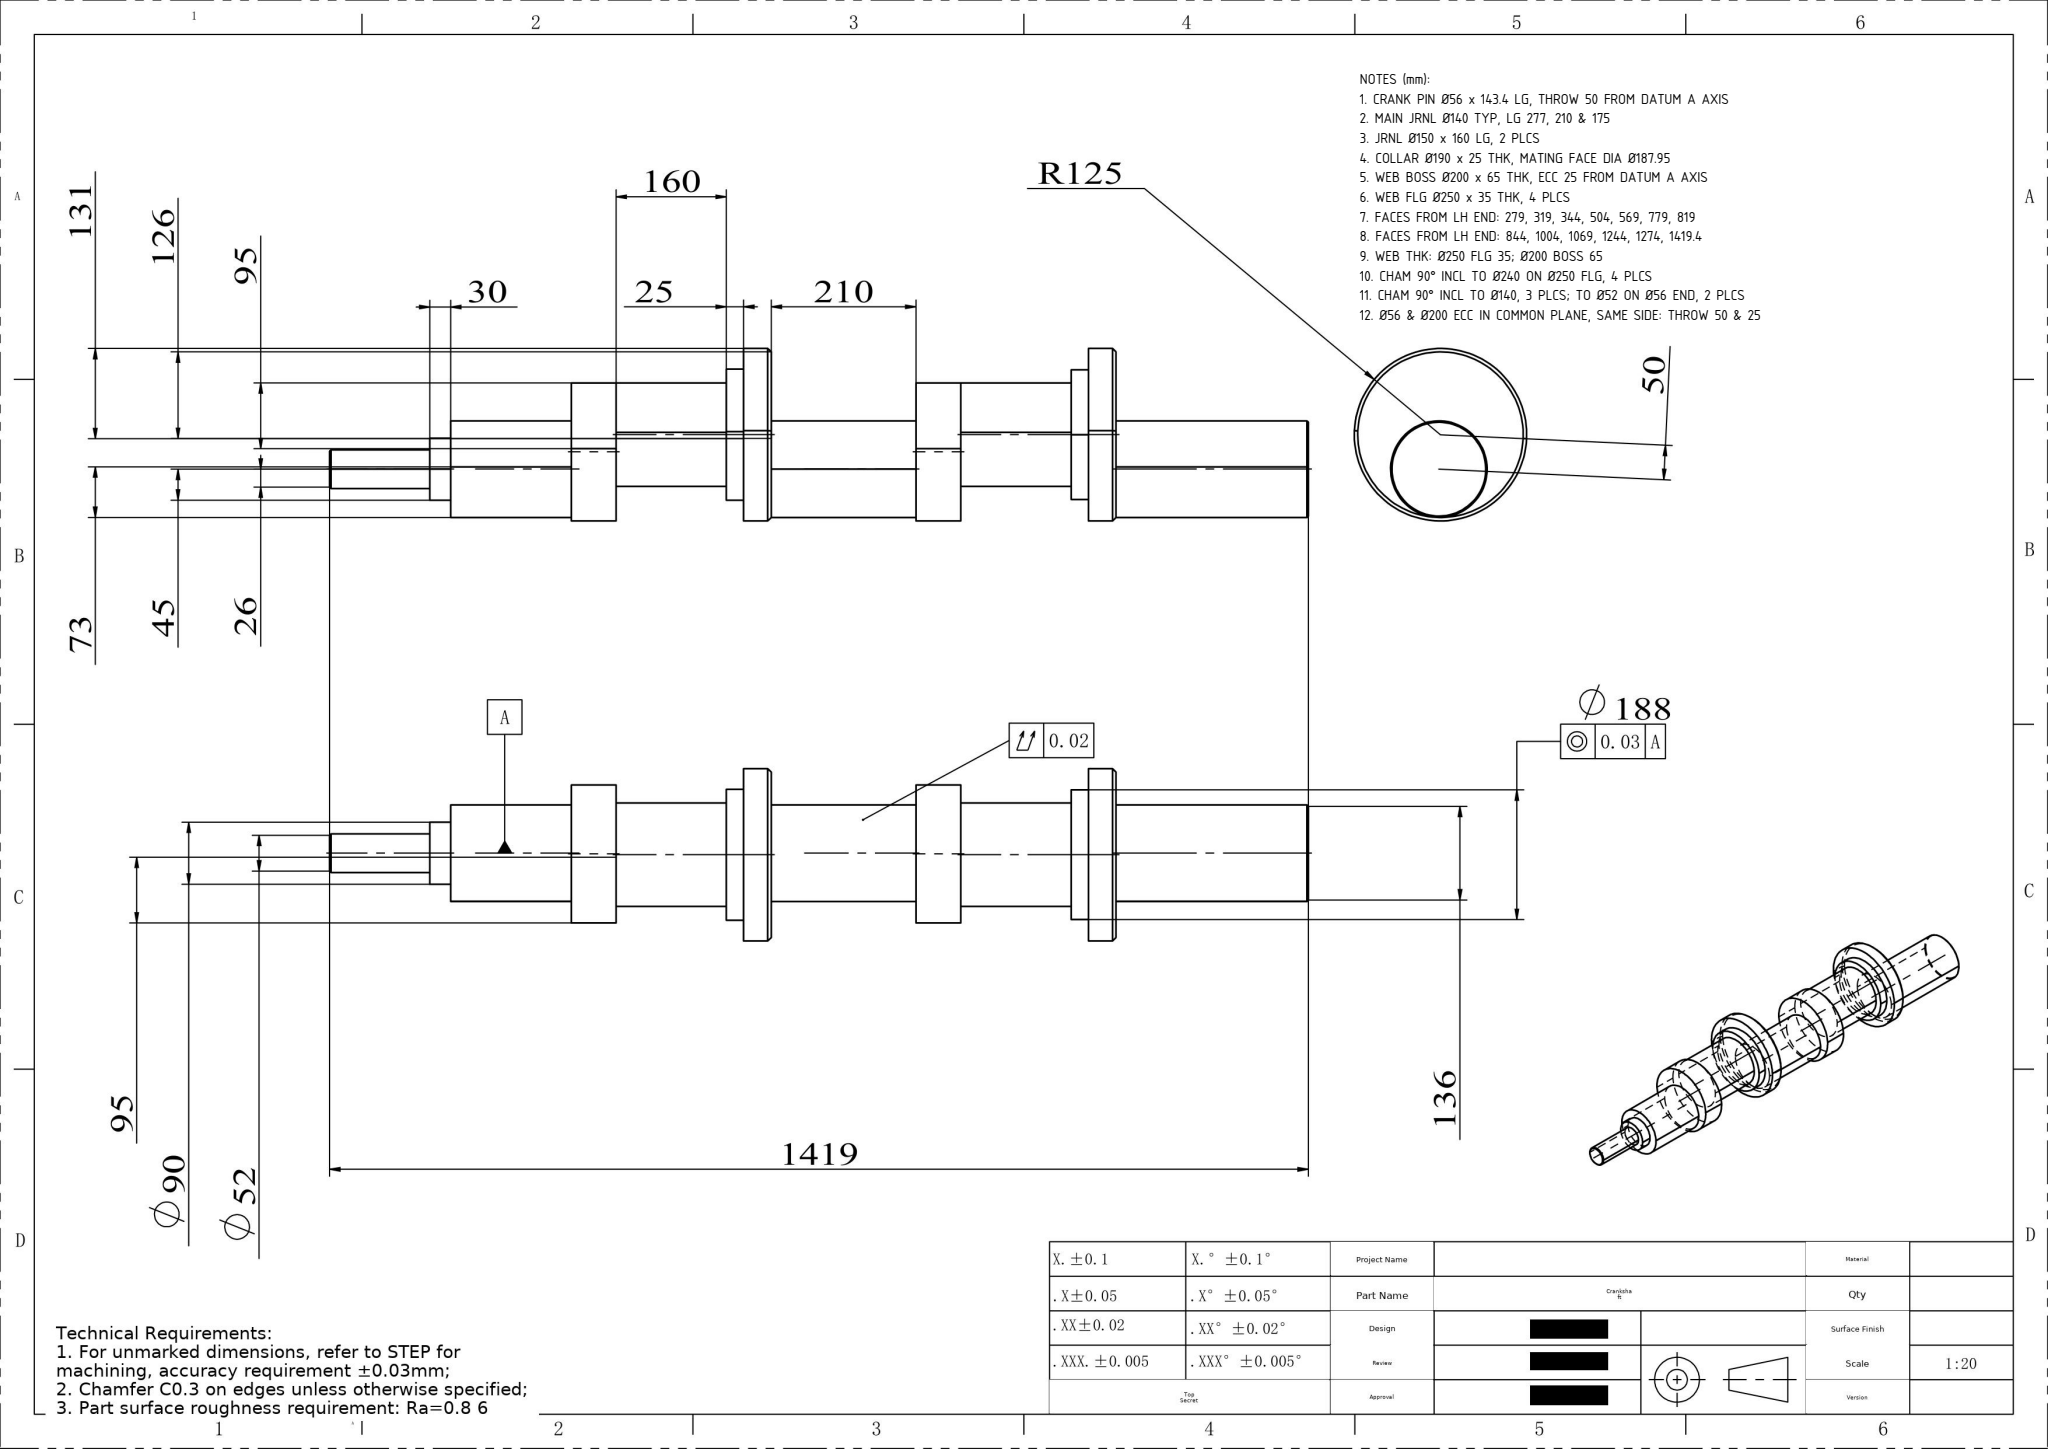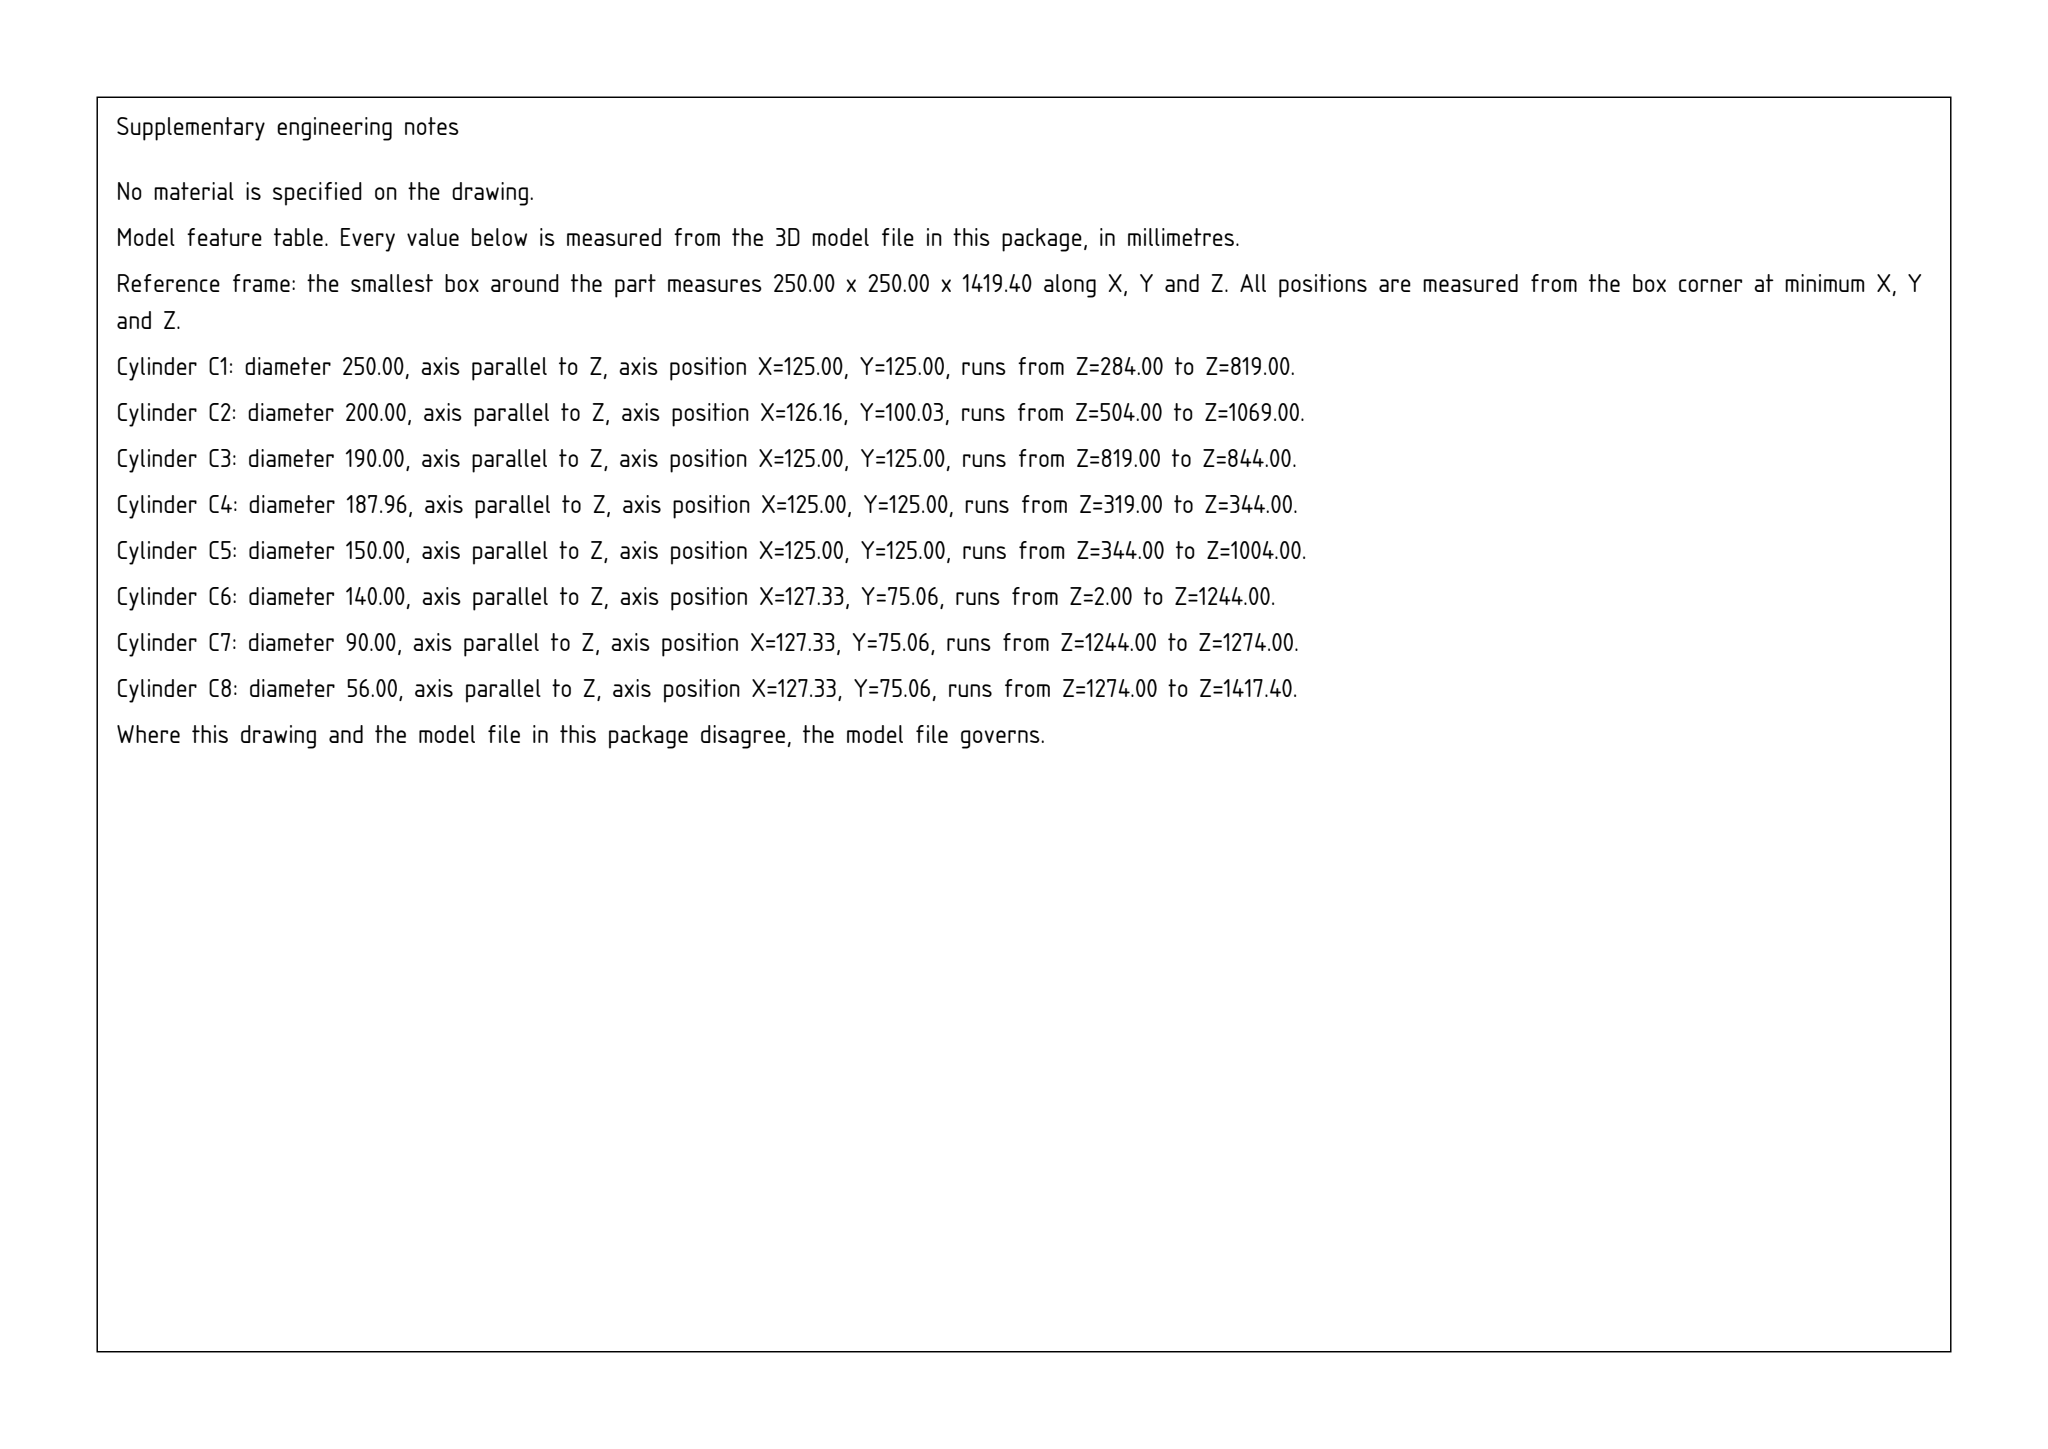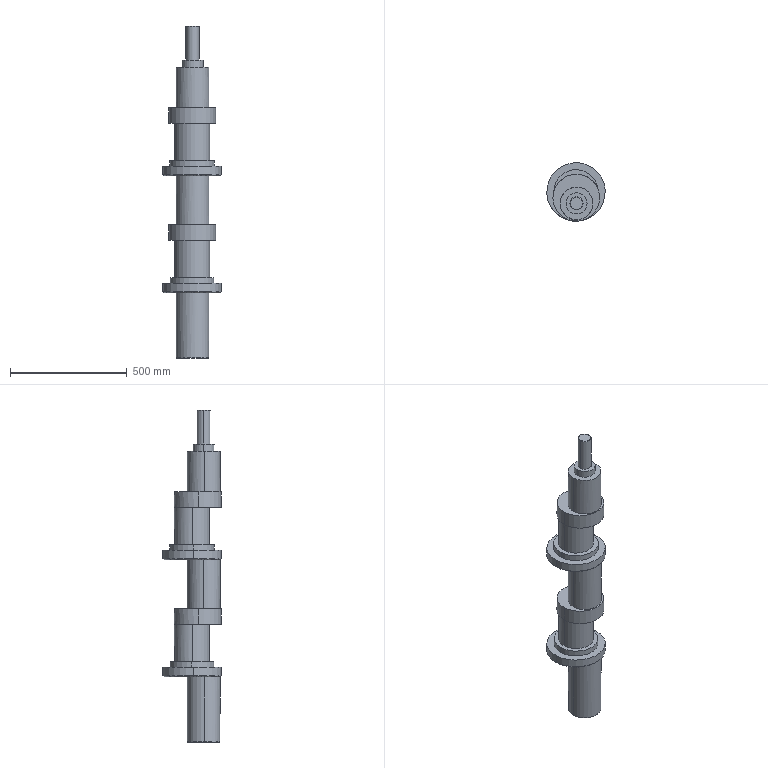Part | SolidWorks | mm | 1 solid | 49 faces | box 250 x 250 x 1419.4 mm | volume 25817361 mm3 | cylinder 26 | plane 14 | cone 9 | commonest cylinder face diameters 140 x6 150 x4 200 x4 250 x4 90 x2 56 x2 187.954 x2 190 x2
Drawing notes:
CRANK PIN Ø56 x 143.4 LG, THROW 50 FROM DATUM A AXIS | from the solid: cyl [56,z,(127.33,75.06),143.4]; offset from axis (125,125) = 50.0
MAIN JRNL Ø140 TYP, LG 277, 210 & 175 | from the solid: cyl [140,z,(127.33,75.06),277/210/175]
JRNL Ø150 x 160 LG, 2 PLCS | from the solid: cyl [150,z,(125,125),160]
COLLAR Ø190 x 25 THK, MATING FACE DIA Ø187.95 | from the solid: cyl [190,z,(125,125),25] & [187.954,z,(125,125),25]
WEB BOSS Ø200 x 65 THK, ECC 25 FROM DATUM A AXIS | from the solid: cyl [200,z,(126.17,100.03),65]; offset from (125,125) = 25.0
WEB FLG Ø250 x 35 THK, 4 PLCS | from the solid: cyl [250,z,(125,125),35] x4
FACES FROM LH END: 279, 319, 344, 504, 569, 779, 819 | from the solid: axis_planes z = 279,319,344,504,569,779,819
FACES FROM LH END: 844, 1004, 1069, 1244, 1274, 1419.4 | from the solid: axis_planes z = 844,1004,1069,1244,1274,1419.4; bbox z 1419.402
WEB THK: Ø250 FLG 35; Ø200 BOSS 65 | from the solid: cyl lengths 35 (Ø250) and 65 (Ø200)
CHAM 90° INCL TO Ø240 ON Ø250 FLG, 4 PLCS | from the solid: cones [90°, ref dia 240, 4] on Ø250 cyls
CHAM 90° INCL TO Ø140, 3 PLCS; TO Ø52 ON Ø56 END, 2 PLCS | from the solid: cones [90°,140,3] and [90°,52,2]
Ø56 & Ø200 ECC IN COMMON PLANE, SAME SIDE: THROW 50 & 25 | from the solid: axes (127.33,75.06) & (126.17,100.03) both offset in same direction from (125,125)